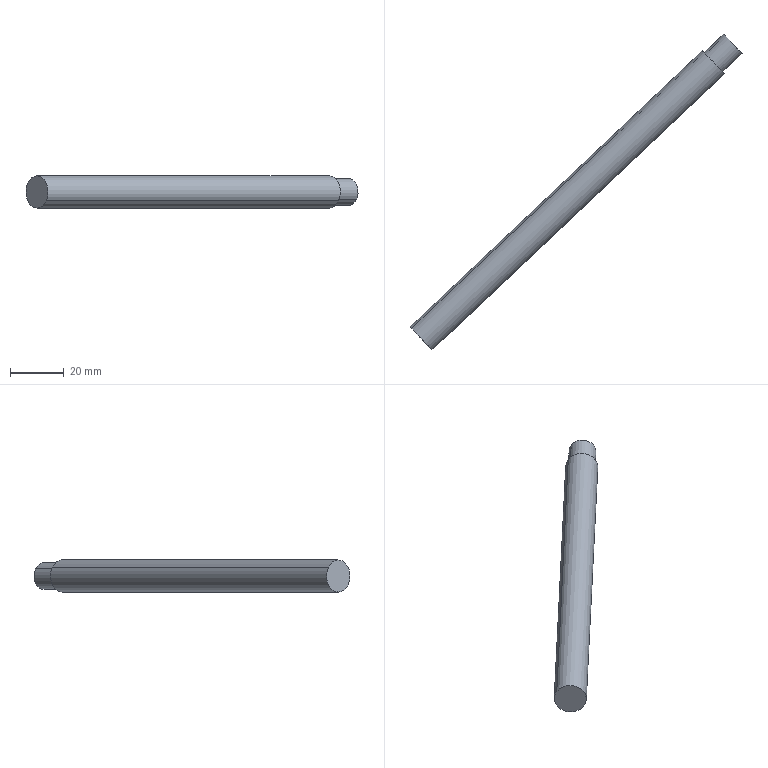Component | SolidWorks | ClampingMechanism-1_LeadScrew-1 | 1 solid | 7 faces | box 123.87 x 117.86 x 12 mm | volume 17750 mm3 | cylinder 4 | plane 3 | commonest cylinder face diameters 10 x2 12 x2
build123d program:
from build123d import *

# Parameters (mm, degrees)
SKETCH1_R           = 6
BOSS_EXTRUDE1_DEPTH = 150
SKETCH2_R           = 5
BOSS_EXTRUDE2_DEPTH = 10


with BuildPart() as part:
    # Sketch1 → Boss-Extrude1 (new body)
    with BuildSketch(Plane.XY):
        Circle(SKETCH1_R)
    extrude(amount=BOSS_EXTRUDE1_DEPTH)

    # Sketch2 → Boss-Extrude2 (add)
    with BuildSketch(Plane(origin=(0, 0, 0), x_dir=(-1, 0, 0), z_dir=(0, 0, -1))):
        Circle(SKETCH2_R)
    extrude(amount=BOSS_EXTRUDE2_DEPTH)


solid = part.part

# Placed as in the assembly
solid = solid.moved(Location((-332.252, -204.3, -542.97), (90, -46.637, 135.815)))
STEP:
#1=COLOUR_RGB('',0.7922,0.8196,0.9333);
#2=FILL_AREA_STYLE_COLOUR('',#1);
#3=FILL_AREA_STYLE('',(#2));
#4=SURFACE_STYLE_FILL_AREA(#3);
#5=SURFACE_SIDE_STYLE('',(#4));
#6=SURFACE_STYLE_USAGE(.BOTH.,#5);
#7=PRESENTATION_STYLE_ASSIGNMENT((#6));
#8=CARTESIAN_POINT('',(-12.681,-7.893,-21.484));
#9=VERTEX_POINT('',#8);
#10=CARTESIAN_POINT('',(-12.908,-7.653,-21.269));
#11=VERTEX_POINT('',#10);
#12=CARTESIAN_POINT('',(-12.795,-7.773,-21.377));
#13=DIRECTION('',(0.727,0.6866,-0.));
#14=DIRECTION('',(0.5747,-0.6085,-0.5472));
#15=AXIS2_PLACEMENT_3D('',#12,#13,#14);
#16=CIRCLE('',#15,0.1969);
#17=EDGE_CURVE('',#9,#11,#16,.T.);
#18=ORIENTED_EDGE('',*,*,#17,.F.);
#19=CARTESIAN_POINT('',(-12.968,-8.163,-21.484));
#20=VERTEX_POINT('',#19);
#21=CARTESIAN_POINT('',(-12.681,-7.893,-21.484));
#22=DIRECTION('',(-0.727,-0.6866,0.));
#23=VECTOR('',#22,39.37);
#24=LINE('',#21,#23);
#25=EDGE_CURVE('',#9,#20,#24,.T.);
#26=ORIENTED_EDGE('',*,*,#25,.T.);
#27=CARTESIAN_POINT('',(-13.194,-7.924,-21.269));
#28=VERTEX_POINT('',#27);
#29=CARTESIAN_POINT('',(-13.081,-8.043,-21.377));
#30=DIRECTION('',(0.727,0.6866,-0.));
#31=DIRECTION('',(0.5747,-0.6085,-0.5472));
#32=AXIS2_PLACEMENT_3D('',#29,#30,#31);
#33=CIRCLE('',#32,0.1969);
#34=EDGE_CURVE('',#20,#28,#33,.T.);
#35=ORIENTED_EDGE('',*,*,#34,.T.);
#36=CARTESIAN_POINT('',(-12.908,-7.653,-21.269));
#37=DIRECTION('',(-0.727,-0.6866,0.));
#38=VECTOR('',#37,39.37);
#39=LINE('',#36,#38);
#40=EDGE_CURVE('',#11,#28,#39,.T.);
#41=ORIENTED_EDGE('',*,*,#40,.F.);
#42=EDGE_LOOP('',(#18,#26,#35,#41));
#43=FACE_OUTER_BOUND('',#42,.T.);
#44=CARTESIAN_POINT('',(-12.795,-7.773,-21.377));
#45=DIRECTION('',(-0.727,-0.6866,0.));
#46=DIRECTION('',(-0.5747,0.6085,0.5472));
#47=AXIS2_PLACEMENT_3D('',#44,#45,#46);
#48=CYLINDRICAL_SURFACE('',#47,0.1969);
#49=ADVANCED_FACE('',(#43),#48,.T.);
#50=CARTESIAN_POINT('',(-17.51,-11.954,-21.247));
#51=VERTEX_POINT('',#50);
#52=CARTESIAN_POINT('',(-17.238,-12.242,-21.506));
#53=VERTEX_POINT('',#52);
#54=CARTESIAN_POINT('',(-17.374,-12.098,-21.377));
#55=DIRECTION('',(-0.727,-0.6866,0.));
#56=DIRECTION('',(-0.5747,0.6085,0.5472));
#57=AXIS2_PLACEMENT_3D('',#54,#55,#56);
#58=CIRCLE('',#57,0.2362);
#59=EDGE_CURVE('',#51,#53,#58,.T.);
#60=ORIENTED_EDGE('',*,*,#59,.F.);
#61=CARTESIAN_POINT('',(-13.217,-7.9,-21.247));
#62=VERTEX_POINT('',#61);
#63=CARTESIAN_POINT('',(-17.51,-11.954,-21.247));
#64=DIRECTION('',(0.727,0.6866,-0.));
#65=VECTOR('',#64,39.37);
#66=LINE('',#63,#65);
#67=EDGE_CURVE('',#51,#62,#66,.T.);
#68=ORIENTED_EDGE('',*,*,#67,.T.);
#69=CARTESIAN_POINT('',(-12.945,-8.187,-21.506));
#70=VERTEX_POINT('',#69);
#71=CARTESIAN_POINT('',(-13.081,-8.043,-21.377));
#72=DIRECTION('',(-0.727,-0.6866,0.));
#73=DIRECTION('',(-0.5747,0.6085,0.5472));
#74=AXIS2_PLACEMENT_3D('',#71,#72,#73);
#75=CIRCLE('',#74,0.2362);
#76=EDGE_CURVE('',#62,#70,#75,.T.);
#77=ORIENTED_EDGE('',*,*,#76,.T.);
#78=CARTESIAN_POINT('',(-17.238,-12.242,-21.506));
#79=DIRECTION('',(0.727,0.6866,-0.));
#80=VECTOR('',#79,39.37);
#81=LINE('',#78,#80);
#82=EDGE_CURVE('',#53,#70,#81,.T.);
#83=ORIENTED_EDGE('',*,*,#82,.F.);
#84=EDGE_LOOP('',(#60,#68,#77,#83));
#85=FACE_OUTER_BOUND('',#84,.T.);
#86=CARTESIAN_POINT('',(-17.374,-12.098,-21.377));
#87=DIRECTION('',(0.727,0.6866,-0.));
#88=DIRECTION('',(0.5747,-0.6085,-0.5472));
#89=AXIS2_PLACEMENT_3D('',#86,#87,#88);
#90=CYLINDRICAL_SURFACE('',#89,0.2362);
#91=ADVANCED_FACE('',(#85),#90,.T.);
#92=ORIENTED_EDGE('',*,*,#67,.F.);
#93=CARTESIAN_POINT('',(-17.374,-12.098,-21.377));
#94=DIRECTION('',(-0.727,-0.6866,0.));
#95=DIRECTION('',(-0.5747,0.6085,0.5472));
#96=AXIS2_PLACEMENT_3D('',#93,#94,#95);
#97=CIRCLE('',#96,0.2362);
#98=EDGE_CURVE('',#53,#51,#97,.T.);
#99=ORIENTED_EDGE('',*,*,#98,.F.);
#100=ORIENTED_EDGE('',*,*,#82,.T.);
#101=CARTESIAN_POINT('',(-13.081,-8.043,-21.377));
#102=DIRECTION('',(-0.727,-0.6866,0.));
#103=DIRECTION('',(-0.5747,0.6085,0.5472));
#104=AXIS2_PLACEMENT_3D('',#101,#102,#103);
#105=CIRCLE('',#104,0.2362);
#106=EDGE_CURVE('',#70,#62,#105,.T.);
#107=ORIENTED_EDGE('',*,*,#106,.T.);
#108=EDGE_LOOP('',(#92,#99,#100,#107));
#109=FACE_OUTER_BOUND('',#108,.T.);
#110=CARTESIAN_POINT('',(-17.374,-12.098,-21.377));
#111=DIRECTION('',(0.727,0.6866,-0.));
#112=DIRECTION('',(0.5747,-0.6085,-0.5472));
#113=AXIS2_PLACEMENT_3D('',#110,#111,#112);
#114=CYLINDRICAL_SURFACE('',#113,0.2362);
#115=ADVANCED_FACE('',(#109),#114,.T.);
#116=ORIENTED_EDGE('',*,*,#98,.T.);
#117=ORIENTED_EDGE('',*,*,#59,.T.);
#118=EDGE_LOOP('',(#116,#117));
#119=FACE_OUTER_BOUND('',#118,.T.);
#120=CARTESIAN_POINT('',(-17.374,-12.098,-21.377));
#121=DIRECTION('',(-0.727,-0.6866,0.));
#122=DIRECTION('',(-0.5747,0.6085,0.5472));
#123=AXIS2_PLACEMENT_3D('',#120,#121,#122);
#124=PLANE('',#123);
#125=ADVANCED_FACE('',(#119),#124,.T.);
#126=CARTESIAN_POINT('',(-13.081,-8.043,-21.377));
#127=DIRECTION('',(0.727,0.6866,-0.));
#128=DIRECTION('',(0.5747,-0.6085,-0.5472));
#129=AXIS2_PLACEMENT_3D('',#126,#127,#128);
#130=CIRCLE('',#129,0.1969);
#131=EDGE_CURVE('',#28,#20,#130,.T.);
#132=ORIENTED_EDGE('',*,*,#131,.F.);
#133=ORIENTED_EDGE('',*,*,#34,.F.);
#134=EDGE_LOOP('',(#132,#133));
#135=FACE_BOUND('',#134,.T.);
#136=ORIENTED_EDGE('',*,*,#106,.F.);
#137=ORIENTED_EDGE('',*,*,#76,.F.);
#138=EDGE_LOOP('',(#136,#137));
#139=FACE_OUTER_BOUND('',#138,.T.);
#140=CARTESIAN_POINT('',(-13.081,-8.043,-21.377));
#141=DIRECTION('',(-0.727,-0.6866,0.));
#142=DIRECTION('',(-0.5747,0.6085,0.5472));
#143=AXIS2_PLACEMENT_3D('',#140,#141,#142);
#144=PLANE('',#143);
#145=ADVANCED_FACE('',(#135,#139),#144,.F.);
#146=ORIENTED_EDGE('',*,*,#25,.F.);
#147=CARTESIAN_POINT('',(-12.795,-7.773,-21.377));
#148=DIRECTION('',(0.727,0.6866,-0.));
#149=DIRECTION('',(0.5747,-0.6085,-0.5472));
#150=AXIS2_PLACEMENT_3D('',#147,#148,#149);
#151=CIRCLE('',#150,0.1969);
#152=EDGE_CURVE('',#11,#9,#151,.T.);
#153=ORIENTED_EDGE('',*,*,#152,.F.);
#154=ORIENTED_EDGE('',*,*,#40,.T.);
#155=ORIENTED_EDGE('',*,*,#131,.T.);
#156=EDGE_LOOP('',(#146,#153,#154,#155));
#157=FACE_OUTER_BOUND('',#156,.T.);
#158=CARTESIAN_POINT('',(-12.795,-7.773,-21.377));
#159=DIRECTION('',(-0.727,-0.6866,0.));
#160=DIRECTION('',(-0.5747,0.6085,0.5472));
#161=AXIS2_PLACEMENT_3D('',#158,#159,#160);
#162=CYLINDRICAL_SURFACE('',#161,0.1969);
#163=ADVANCED_FACE('',(#157),#162,.T.);
#164=ORIENTED_EDGE('',*,*,#152,.T.);
#165=ORIENTED_EDGE('',*,*,#17,.T.);
#166=EDGE_LOOP('',(#164,#165));
#167=FACE_OUTER_BOUND('',#166,.T.);
#168=CARTESIAN_POINT('',(-12.795,-7.773,-21.377));
#169=DIRECTION('',(0.727,0.6866,-0.));
#170=DIRECTION('',(0.5747,-0.6085,-0.5472));
#171=AXIS2_PLACEMENT_3D('',#168,#169,#170);
#172=PLANE('',#171);
#173=ADVANCED_FACE('',(#167),#172,.T.);
#174=CLOSED_SHELL('',(#49,#91,#115,#125,#145,#163,#173));
#175=MANIFOLD_SOLID_BREP('',#174);
#176=STYLED_ITEM('',(#7),#175);
#177=PRESENTATION_LAYER_ASSIGNMENT('','',(#176));
#178=(LENGTH_UNIT()NAMED_UNIT(*)SI_UNIT($,.METRE.));
#179=LENGTH_MEASURE_WITH_UNIT(LENGTH_MEASURE(0.0254),#178);
#180=DIMENSIONAL_EXPONENTS(1.,0.,0.,0.,0.,0.,0.);
#181=(CONVERSION_BASED_UNIT('',#179)LENGTH_UNIT()NAMED_UNIT(#180));
#182=UNCERTAINTY_MEASURE_WITH_UNIT(LENGTH_MEASURE(0.00001),#181,'','');
#183=(NAMED_UNIT(*)PLANE_ANGLE_UNIT()SI_UNIT($,.RADIAN.));
#184=(NAMED_UNIT(*)SI_UNIT($,.STERADIAN.)SOLID_ANGLE_UNIT());
#185=(GEOMETRIC_REPRESENTATION_CONTEXT(3)GLOBAL_UNCERTAINTY_ASSIGNED_CONTEXT((#182))GLOBAL_UNIT_ASSIGNED_CONTEXT((#181,#183,#184))REPRESENTATION_CONTEXT('',''));
#186=MECHANICAL_DESIGN_GEOMETRIC_PRESENTATION_REPRESENTATION('',(#176),#185);
#187=CARTESIAN_POINT('',(0.,0.,0.));
#188=DIRECTION('',(0.,0.,1.));
#189=DIRECTION('',(1.,0.,0.));
#190=AXIS2_PLACEMENT_3D('',#187,#188,#189);
#191=(LENGTH_UNIT()NAMED_UNIT(*)SI_UNIT($,.METRE.));
#192=LENGTH_MEASURE_WITH_UNIT(LENGTH_MEASURE(0.0254),#191);
#193=DIMENSIONAL_EXPONENTS(1.,0.,0.,0.,0.,0.,0.);
#194=(CONVERSION_BASED_UNIT('',#192)LENGTH_UNIT()NAMED_UNIT(#193));
#195=UNCERTAINTY_MEASURE_WITH_UNIT(LENGTH_MEASURE(0.00001),#194,'','');
#196=(NAMED_UNIT(*)PLANE_ANGLE_UNIT()SI_UNIT($,.RADIAN.));
#197=(NAMED_UNIT(*)SI_UNIT($,.STERADIAN.)SOLID_ANGLE_UNIT());
#198=(GEOMETRIC_REPRESENTATION_CONTEXT(3)GLOBAL_UNCERTAINTY_ASSIGNED_CONTEXT((#195))GLOBAL_UNIT_ASSIGNED_CONTEXT((#194,#196,#197))REPRESENTATION_CONTEXT('',''));
#199=ADVANCED_BREP_SHAPE_REPRESENTATION('',(#175,#190),#198);